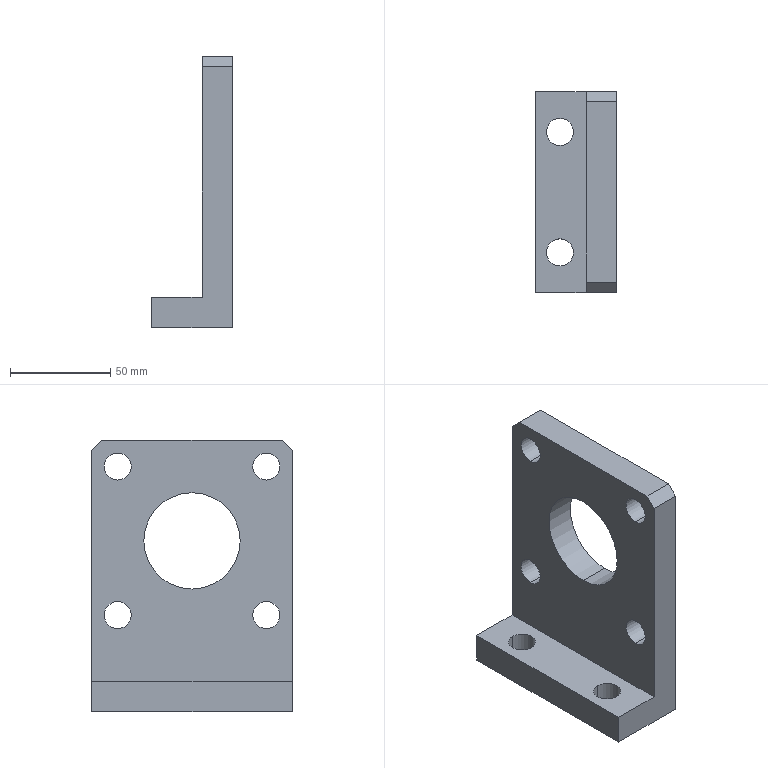Component | SolidWorks | ZN-A-012-1 | 1 solid | 24 faces | box 40 x 100 x 135 mm | volume 199599 mm3 | cylinder 14 | plane 10 | commonest cylinder face diameters 13.5 x12 48 x2
build123d program:
from build123d import *

# Parameters (mm, degrees)
SKETCH1_W                 = 100
SKETCH1_H                 = 135
BOSS_EXTRUDE1_DEPTH       = 7.5
SKETCH2_W                 = 15
SKETCH2_H                 = 25
BOSS_EXTRUDE2_DEPTH       = 100
SKETCH3_R                 = 24
CUT_EXTRUDE1_DEPTH        = 94.039
M12_CLEARANCE_HOLE1_D     = 13.5
M12_CLEARANCE_HOLE1_DEPTH = 15
M12_CLEARANCE_HOLE1_TIP   = 4.056
M12_CLEARANCE_HOLE2_D     = 13.5
M12_CLEARANCE_HOLE2_DEPTH = 15
M12_CLEARANCE_HOLE2_TIP   = 4.056
CHAMFER1_SIZE             = 5


with BuildPart() as part:
    # Sketch1 → Boss-Extrude1 (new, symmetric)
    with BuildSketch(Plane(origin=(0, 0, 0), x_dir=(1, 0, 0), z_dir=(0, 1, 0))):
        Rectangle(SKETCH1_W, SKETCH1_H)
    extrude(amount=BOSS_EXTRUDE1_DEPTH, both=True)

    # Sketch2 → Boss-Extrude2 (add)
    with BuildSketch(Plane.ZY.offset(50)):
        with Locations((60, 20)):
            Rectangle(SKETCH2_W, SKETCH2_H)
    extrude(amount=-BOSS_EXTRUDE2_DEPTH)

    # Sketch3 → Cut-Extrude1 (cut, through all)
    with BuildSketch(Plane.XZ.offset(7.5)):
        with Locations(Location((0, -17.5, 0), (0, 0, 270))):
            Circle(SKETCH3_R)
    extrude(amount=-CUT_EXTRUDE1_DEPTH, mode=Mode.SUBTRACT)

    # M12 Clearance Hole1
    with Locations(Plane(origin=(0, 7.5, 0), x_dir=(1, 0, 0), z_dir=(0, 1, 0))):
        with Locations((-37, 54.5), (37, 54.5), (-37, -19.5), (37, -19.5)):
            Hole(M12_CLEARANCE_HOLE1_D / 2, depth=M12_CLEARANCE_HOLE1_DEPTH)
            with Locations((0, 0, -(M12_CLEARANCE_HOLE1_DEPTH + M12_CLEARANCE_HOLE1_TIP / 2))):  # 118° drill point
                Cone(0, M12_CLEARANCE_HOLE1_D / 2, M12_CLEARANCE_HOLE1_TIP, mode=Mode.SUBTRACT)

    # M12 Clearance Hole2
    with Locations(Plane(origin=(0, 0, 52.5), x_dir=(-1, 0, 0), z_dir=(0, 0, -1))):
        with Locations((-30, 20.5), (30, 20.5)):
            Hole(M12_CLEARANCE_HOLE2_D / 2, depth=M12_CLEARANCE_HOLE2_DEPTH)
            with Locations((0, 0, -(M12_CLEARANCE_HOLE2_DEPTH + M12_CLEARANCE_HOLE2_TIP / 2))):  # 118° drill point
                Cone(0, M12_CLEARANCE_HOLE2_D / 2, M12_CLEARANCE_HOLE2_TIP, mode=Mode.SUBTRACT)

    # Chamfer1
    chamfer1_edges = [part.edges().sort_by_distance(p)[0] for p in [
        (50, 0, -67.5),
        (-50, 0, -67.5),
    ]]
    chamfer(chamfer1_edges, length=CHAMFER1_SIZE)


solid = part.part

# Placed as in the assembly
solid = solid.moved(Location((640.892, 232.499, 82.5), (180, 0, 90)))
STEP:
#1=CARTESIAN_POINT('',(24.425,7.707,0.5906));
#2=VERTEX_POINT('',#1);
#3=CARTESIAN_POINT('',(24.425,8.238,0.5906));
#4=VERTEX_POINT('',#3);
#5=CARTESIAN_POINT('',(24.425,7.972,0.5906));
#6=DIRECTION('',(-0.,-0.,1.));
#7=DIRECTION('',(0.,1.,0.));
#8=AXIS2_PLACEMENT_3D('',#5,#6,#7);
#9=CIRCLE('',#8,0.2657);
#10=EDGE_CURVE('',#2,#4,#9,.T.);
#11=ORIENTED_EDGE('',*,*,#10,.F.);
#12=CARTESIAN_POINT('',(24.425,7.707,1.181));
#13=VERTEX_POINT('',#12);
#14=CARTESIAN_POINT('',(24.425,7.707,1.181));
#15=DIRECTION('',(-0.,-0.,1.));
#16=VECTOR('',#15,39.37);
#17=LINE('',#14,#16);
#18=EDGE_CURVE('',#2,#13,#17,.T.);
#19=ORIENTED_EDGE('',*,*,#18,.T.);
#20=CARTESIAN_POINT('',(24.425,8.238,1.181));
#21=VERTEX_POINT('',#20);
#22=CARTESIAN_POINT('',(24.425,7.972,1.181));
#23=DIRECTION('',(-0.,-0.,1.));
#24=DIRECTION('',(0.,1.,0.));
#25=AXIS2_PLACEMENT_3D('',#22,#23,#24);
#26=CIRCLE('',#25,0.2657);
#27=EDGE_CURVE('',#13,#21,#26,.T.);
#28=ORIENTED_EDGE('',*,*,#27,.T.);
#29=CARTESIAN_POINT('',(24.425,8.238,1.181));
#30=DIRECTION('',(-0.,-0.,1.));
#31=VECTOR('',#30,39.37);
#32=LINE('',#29,#31);
#33=EDGE_CURVE('',#4,#21,#32,.T.);
#34=ORIENTED_EDGE('',*,*,#33,.F.);
#35=EDGE_LOOP('',(#11,#19,#28,#34));
#36=FACE_OUTER_BOUND('',#35,.T.);
#37=CARTESIAN_POINT('',(24.425,7.972,1.181));
#38=DIRECTION('',(-0.,-0.,1.));
#39=DIRECTION('',(0.,1.,0.));
#40=AXIS2_PLACEMENT_3D('',#37,#38,#39);
#41=CYLINDRICAL_SURFACE('',#40,0.2657);
#42=ADVANCED_FACE('',(#36),#41,.F.);
#43=CARTESIAN_POINT('',(24.425,10.069,0.5906));
#44=VERTEX_POINT('',#43);
#45=CARTESIAN_POINT('',(24.425,10.6,0.5906));
#46=VERTEX_POINT('',#45);
#47=CARTESIAN_POINT('',(24.425,10.335,0.5906));
#48=DIRECTION('',(-0.,-0.,1.));
#49=DIRECTION('',(0.,1.,0.));
#50=AXIS2_PLACEMENT_3D('',#47,#48,#49);
#51=CIRCLE('',#50,0.2657);
#52=EDGE_CURVE('',#44,#46,#51,.T.);
#53=ORIENTED_EDGE('',*,*,#52,.F.);
#54=CARTESIAN_POINT('',(24.425,10.069,1.181));
#55=VERTEX_POINT('',#54);
#56=CARTESIAN_POINT('',(24.425,10.069,1.181));
#57=DIRECTION('',(-0.,-0.,1.));
#58=VECTOR('',#57,39.37);
#59=LINE('',#56,#58);
#60=EDGE_CURVE('',#44,#55,#59,.T.);
#61=ORIENTED_EDGE('',*,*,#60,.T.);
#62=CARTESIAN_POINT('',(24.425,10.6,1.181));
#63=VERTEX_POINT('',#62);
#64=CARTESIAN_POINT('',(24.425,10.335,1.181));
#65=DIRECTION('',(-0.,-0.,1.));
#66=DIRECTION('',(0.,1.,0.));
#67=AXIS2_PLACEMENT_3D('',#64,#65,#66);
#68=CIRCLE('',#67,0.2657);
#69=EDGE_CURVE('',#55,#63,#68,.T.);
#70=ORIENTED_EDGE('',*,*,#69,.T.);
#71=CARTESIAN_POINT('',(24.425,10.6,1.181));
#72=DIRECTION('',(-0.,-0.,1.));
#73=VECTOR('',#72,39.37);
#74=LINE('',#71,#73);
#75=EDGE_CURVE('',#46,#63,#74,.T.);
#76=ORIENTED_EDGE('',*,*,#75,.F.);
#77=EDGE_LOOP('',(#53,#61,#70,#76));
#78=FACE_OUTER_BOUND('',#77,.T.);
#79=CARTESIAN_POINT('',(24.425,10.335,1.181));
#80=DIRECTION('',(-0.,-0.,1.));
#81=DIRECTION('',(0.,1.,0.));
#82=AXIS2_PLACEMENT_3D('',#79,#80,#81);
#83=CYLINDRICAL_SURFACE('',#82,0.2657);
#84=ADVANCED_FACE('',(#78),#83,.F.);
#85=CARTESIAN_POINT('',(25.527,10.61,5.659));
#86=VERTEX_POINT('',#85);
#87=CARTESIAN_POINT('',(25.527,10.61,5.128));
#88=VERTEX_POINT('',#87);
#89=CARTESIAN_POINT('',(25.527,10.61,5.394));
#90=DIRECTION('',(-1.,-0.,-0.));
#91=DIRECTION('',(0.,0.,-1.));
#92=AXIS2_PLACEMENT_3D('',#89,#90,#91);
#93=CIRCLE('',#92,0.2657);
#94=EDGE_CURVE('',#86,#88,#93,.T.);
#95=ORIENTED_EDGE('',*,*,#94,.F.);
#96=CARTESIAN_POINT('',(24.937,10.61,5.659));
#97=VERTEX_POINT('',#96);
#98=CARTESIAN_POINT('',(24.937,10.61,5.659));
#99=DIRECTION('',(-1.,-0.,-0.));
#100=VECTOR('',#99,39.37);
#101=LINE('',#98,#100);
#102=EDGE_CURVE('',#86,#97,#101,.T.);
#103=ORIENTED_EDGE('',*,*,#102,.T.);
#104=CARTESIAN_POINT('',(24.937,10.61,5.128));
#105=VERTEX_POINT('',#104);
#106=CARTESIAN_POINT('',(24.937,10.61,5.394));
#107=DIRECTION('',(-1.,-0.,-0.));
#108=DIRECTION('',(0.,0.,-1.));
#109=AXIS2_PLACEMENT_3D('',#106,#107,#108);
#110=CIRCLE('',#109,0.2657);
#111=EDGE_CURVE('',#97,#105,#110,.T.);
#112=ORIENTED_EDGE('',*,*,#111,.T.);
#113=CARTESIAN_POINT('',(24.937,10.61,5.128));
#114=DIRECTION('',(-1.,-0.,-0.));
#115=VECTOR('',#114,39.37);
#116=LINE('',#113,#115);
#117=EDGE_CURVE('',#88,#105,#116,.T.);
#118=ORIENTED_EDGE('',*,*,#117,.F.);
#119=EDGE_LOOP('',(#95,#103,#112,#118));
#120=FACE_OUTER_BOUND('',#119,.T.);
#121=CARTESIAN_POINT('',(24.937,10.61,5.394));
#122=DIRECTION('',(-1.,-0.,-0.));
#123=DIRECTION('',(0.,0.,-1.));
#124=AXIS2_PLACEMENT_3D('',#121,#122,#123);
#125=CYLINDRICAL_SURFACE('',#124,0.2657);
#126=ADVANCED_FACE('',(#120),#125,.F.);
#127=CARTESIAN_POINT('',(25.527,7.697,5.659));
#128=VERTEX_POINT('',#127);
#129=CARTESIAN_POINT('',(25.527,7.697,5.128));
#130=VERTEX_POINT('',#129);
#131=CARTESIAN_POINT('',(25.527,7.697,5.394));
#132=DIRECTION('',(-1.,-0.,-0.));
#133=DIRECTION('',(0.,0.,-1.));
#134=AXIS2_PLACEMENT_3D('',#131,#132,#133);
#135=CIRCLE('',#134,0.2657);
#136=EDGE_CURVE('',#128,#130,#135,.T.);
#137=ORIENTED_EDGE('',*,*,#136,.F.);
#138=CARTESIAN_POINT('',(24.937,7.697,5.659));
#139=VERTEX_POINT('',#138);
#140=CARTESIAN_POINT('',(24.937,7.697,5.659));
#141=DIRECTION('',(-1.,-0.,-0.));
#142=VECTOR('',#141,39.37);
#143=LINE('',#140,#142);
#144=EDGE_CURVE('',#128,#139,#143,.T.);
#145=ORIENTED_EDGE('',*,*,#144,.T.);
#146=CARTESIAN_POINT('',(24.937,7.697,5.128));
#147=VERTEX_POINT('',#146);
#148=CARTESIAN_POINT('',(24.937,7.697,5.394));
#149=DIRECTION('',(-1.,-0.,-0.));
#150=DIRECTION('',(0.,0.,-1.));
#151=AXIS2_PLACEMENT_3D('',#148,#149,#150);
#152=CIRCLE('',#151,0.2657);
#153=EDGE_CURVE('',#139,#147,#152,.T.);
#154=ORIENTED_EDGE('',*,*,#153,.T.);
#155=CARTESIAN_POINT('',(24.937,7.697,5.128));
#156=DIRECTION('',(-1.,-0.,-0.));
#157=VECTOR('',#156,39.37);
#158=LINE('',#155,#157);
#159=EDGE_CURVE('',#130,#147,#158,.T.);
#160=ORIENTED_EDGE('',*,*,#159,.F.);
#161=EDGE_LOOP('',(#137,#145,#154,#160));
#162=FACE_OUTER_BOUND('',#161,.T.);
#163=CARTESIAN_POINT('',(24.937,7.697,5.394));
#164=DIRECTION('',(-1.,-0.,-0.));
#165=DIRECTION('',(0.,0.,-1.));
#166=AXIS2_PLACEMENT_3D('',#163,#164,#165);
#167=CYLINDRICAL_SURFACE('',#166,0.2657);
#168=ADVANCED_FACE('',(#162),#167,.F.);
#169=CARTESIAN_POINT('',(25.527,10.61,2.746));
#170=VERTEX_POINT('',#169);
#171=CARTESIAN_POINT('',(25.527,10.61,2.215));
#172=VERTEX_POINT('',#171);
#173=CARTESIAN_POINT('',(25.527,10.61,2.48));
#174=DIRECTION('',(-1.,-0.,-0.));
#175=DIRECTION('',(0.,0.,-1.));
#176=AXIS2_PLACEMENT_3D('',#173,#174,#175);
#177=CIRCLE('',#176,0.2657);
#178=EDGE_CURVE('',#170,#172,#177,.T.);
#179=ORIENTED_EDGE('',*,*,#178,.F.);
#180=CARTESIAN_POINT('',(24.937,10.61,2.746));
#181=VERTEX_POINT('',#180);
#182=CARTESIAN_POINT('',(24.937,10.61,2.746));
#183=DIRECTION('',(-1.,-0.,-0.));
#184=VECTOR('',#183,39.37);
#185=LINE('',#182,#184);
#186=EDGE_CURVE('',#170,#181,#185,.T.);
#187=ORIENTED_EDGE('',*,*,#186,.T.);
#188=CARTESIAN_POINT('',(24.937,10.61,2.215));
#189=VERTEX_POINT('',#188);
#190=CARTESIAN_POINT('',(24.937,10.61,2.48));
#191=DIRECTION('',(-1.,-0.,-0.));
#192=DIRECTION('',(0.,0.,-1.));
#193=AXIS2_PLACEMENT_3D('',#190,#191,#192);
#194=CIRCLE('',#193,0.2657);
#195=EDGE_CURVE('',#181,#189,#194,.T.);
#196=ORIENTED_EDGE('',*,*,#195,.T.);
#197=CARTESIAN_POINT('',(24.937,10.61,2.215));
#198=DIRECTION('',(-1.,-0.,-0.));
#199=VECTOR('',#198,39.37);
#200=LINE('',#197,#199);
#201=EDGE_CURVE('',#172,#189,#200,.T.);
#202=ORIENTED_EDGE('',*,*,#201,.F.);
#203=EDGE_LOOP('',(#179,#187,#196,#202));
#204=FACE_OUTER_BOUND('',#203,.T.);
#205=CARTESIAN_POINT('',(24.937,10.61,2.48));
#206=DIRECTION('',(-1.,-0.,-0.));
#207=DIRECTION('',(0.,0.,-1.));
#208=AXIS2_PLACEMENT_3D('',#205,#206,#207);
#209=CYLINDRICAL_SURFACE('',#208,0.2657);
#210=ADVANCED_FACE('',(#204),#209,.F.);
#211=CARTESIAN_POINT('',(25.527,7.697,2.746));
#212=VERTEX_POINT('',#211);
#213=CARTESIAN_POINT('',(25.527,7.697,2.215));
#214=VERTEX_POINT('',#213);
#215=CARTESIAN_POINT('',(25.527,7.697,2.48));
#216=DIRECTION('',(-1.,-0.,-0.));
#217=DIRECTION('',(0.,0.,-1.));
#218=AXIS2_PLACEMENT_3D('',#215,#216,#217);
#219=CIRCLE('',#218,0.2657);
#220=EDGE_CURVE('',#212,#214,#219,.T.);
#221=ORIENTED_EDGE('',*,*,#220,.F.);
#222=CARTESIAN_POINT('',(24.937,7.697,2.746));
#223=VERTEX_POINT('',#222);
#224=CARTESIAN_POINT('',(24.937,7.697,2.746));
#225=DIRECTION('',(-1.,-0.,-0.));
#226=VECTOR('',#225,39.37);
#227=LINE('',#224,#226);
#228=EDGE_CURVE('',#212,#223,#227,.T.);
#229=ORIENTED_EDGE('',*,*,#228,.T.);
#230=CARTESIAN_POINT('',(24.937,7.697,2.215));
#231=VERTEX_POINT('',#230);
#232=CARTESIAN_POINT('',(24.937,7.697,2.48));
#233=DIRECTION('',(-1.,-0.,-0.));
#234=DIRECTION('',(0.,0.,-1.));
#235=AXIS2_PLACEMENT_3D('',#232,#233,#234);
#236=CIRCLE('',#235,0.2657);
#237=EDGE_CURVE('',#223,#231,#236,.T.);
#238=ORIENTED_EDGE('',*,*,#237,.T.);
#239=CARTESIAN_POINT('',(24.937,7.697,2.215));
#240=DIRECTION('',(-1.,-0.,-0.));
#241=VECTOR('',#240,39.37);
#242=LINE('',#239,#241);
#243=EDGE_CURVE('',#214,#231,#242,.T.);
#244=ORIENTED_EDGE('',*,*,#243,.F.);
#245=EDGE_LOOP('',(#221,#229,#238,#244));
#246=FACE_OUTER_BOUND('',#245,.T.);
#247=CARTESIAN_POINT('',(24.937,7.697,2.48));
#248=DIRECTION('',(-1.,-0.,-0.));
#249=DIRECTION('',(0.,0.,-1.));
#250=AXIS2_PLACEMENT_3D('',#247,#248,#249);
#251=CYLINDRICAL_SURFACE('',#250,0.2657);
#252=ADVANCED_FACE('',(#246),#251,.F.);
#253=CARTESIAN_POINT('',(24.937,9.154,4.882));
#254=VERTEX_POINT('',#253);
#255=CARTESIAN_POINT('',(24.937,9.154,2.992));
#256=VERTEX_POINT('',#255);
#257=CARTESIAN_POINT('',(24.937,9.154,3.937));
#258=DIRECTION('',(-1.,-0.,-0.));
#259=DIRECTION('',(0.,0.,-1.));
#260=AXIS2_PLACEMENT_3D('',#257,#258,#259);
#261=CIRCLE('',#260,0.9449);
#262=EDGE_CURVE('',#254,#256,#261,.T.);
#263=ORIENTED_EDGE('',*,*,#262,.T.);
#264=CARTESIAN_POINT('',(25.527,9.154,2.992));
#265=VERTEX_POINT('',#264);
#266=CARTESIAN_POINT('',(23.952,9.154,2.992));
#267=DIRECTION('',(1.,0.,0.));
#268=VECTOR('',#267,39.37);
#269=LINE('',#266,#268);
#270=EDGE_CURVE('',#256,#265,#269,.T.);
#271=ORIENTED_EDGE('',*,*,#270,.T.);
#272=CARTESIAN_POINT('',(25.527,9.154,4.882));
#273=VERTEX_POINT('',#272);
#274=CARTESIAN_POINT('',(25.527,9.154,3.937));
#275=DIRECTION('',(1.,0.,0.));
#276=DIRECTION('',(0.,-0.,1.));
#277=AXIS2_PLACEMENT_3D('',#274,#275,#276);
#278=CIRCLE('',#277,0.9449);
#279=EDGE_CURVE('',#265,#273,#278,.T.);
#280=ORIENTED_EDGE('',*,*,#279,.T.);
#281=CARTESIAN_POINT('',(23.952,9.154,4.882));
#282=DIRECTION('',(1.,0.,0.));
#283=VECTOR('',#282,39.37);
#284=LINE('',#281,#283);
#285=EDGE_CURVE('',#254,#273,#284,.T.);
#286=ORIENTED_EDGE('',*,*,#285,.F.);
#287=EDGE_LOOP('',(#263,#271,#280,#286));
#288=FACE_OUTER_BOUND('',#287,.T.);
#289=CARTESIAN_POINT('',(23.952,9.154,3.937));
#290=DIRECTION('',(1.,0.,0.));
#291=DIRECTION('',(0.,-0.,1.));
#292=AXIS2_PLACEMENT_3D('',#289,#290,#291);
#293=CYLINDRICAL_SURFACE('',#292,0.9449);
#294=ADVANCED_FACE('',(#288),#293,.F.);
#295=CARTESIAN_POINT('',(24.937,11.122,5.709));
#296=VERTEX_POINT('',#295);
#297=CARTESIAN_POINT('',(24.937,11.122,1.181));
#298=VERTEX_POINT('',#297);
#299=CARTESIAN_POINT('',(24.937,11.122,5.906));
#300=DIRECTION('',(0.,0.,-1.));
#301=VECTOR('',#300,39.37);
#302=LINE('',#299,#301);
#303=EDGE_CURVE('',#296,#298,#302,.T.);
#304=ORIENTED_EDGE('',*,*,#303,.F.);
#305=CARTESIAN_POINT('',(25.527,11.122,5.709));
#306=VERTEX_POINT('',#305);
#307=CARTESIAN_POINT('',(24.937,11.122,5.709));
#308=DIRECTION('',(1.,0.,0.));
#309=VECTOR('',#308,39.37);
#310=LINE('',#307,#309);
#311=EDGE_CURVE('',#296,#306,#310,.T.);
#312=ORIENTED_EDGE('',*,*,#311,.T.);
#313=CARTESIAN_POINT('',(25.527,11.122,0.5906));
#314=VERTEX_POINT('',#313);
#315=CARTESIAN_POINT('',(25.527,11.122,5.906));
#316=DIRECTION('',(0.,0.,-1.));
#317=VECTOR('',#316,39.37);
#318=LINE('',#315,#317);
#319=EDGE_CURVE('',#306,#314,#318,.T.);
#320=ORIENTED_EDGE('',*,*,#319,.T.);
#321=CARTESIAN_POINT('',(23.952,11.122,0.5906));
#322=VERTEX_POINT('',#321);
#323=CARTESIAN_POINT('',(24.937,11.122,0.5906));
#324=DIRECTION('',(1.,0.,0.));
#325=VECTOR('',#324,39.37);
#326=LINE('',#323,#325);
#327=EDGE_CURVE('',#322,#314,#326,.T.);
#328=ORIENTED_EDGE('',*,*,#327,.F.);
#329=CARTESIAN_POINT('',(23.952,11.122,1.181));
#330=VERTEX_POINT('',#329);
#331=CARTESIAN_POINT('',(23.952,11.122,0.5906));
#332=DIRECTION('',(-0.,-0.,1.));
#333=VECTOR('',#332,39.37);
#334=LINE('',#331,#333);
#335=EDGE_CURVE('',#322,#330,#334,.T.);
#336=ORIENTED_EDGE('',*,*,#335,.T.);
#337=CARTESIAN_POINT('',(24.937,11.122,1.181));
#338=DIRECTION('',(1.,0.,0.));
#339=VECTOR('',#338,39.37);
#340=LINE('',#337,#339);
#341=EDGE_CURVE('',#330,#298,#340,.T.);
#342=ORIENTED_EDGE('',*,*,#341,.T.);
#343=EDGE_LOOP('',(#304,#312,#320,#328,#336,#342));
#344=FACE_OUTER_BOUND('',#343,.T.);
#345=CARTESIAN_POINT('',(24.937,11.122,5.906));
#346=DIRECTION('',(0.,-1.,-0.));
#347=DIRECTION('',(-0.,-0.,1.));
#348=AXIS2_PLACEMENT_3D('',#345,#346,#347);
#349=PLANE('',#348);
#350=ADVANCED_FACE('',(#344),#349,.F.);
#351=CARTESIAN_POINT('',(24.425,7.972,0.5906));
#352=DIRECTION('',(-0.,-0.,1.));
#353=DIRECTION('',(0.,1.,0.));
#354=AXIS2_PLACEMENT_3D('',#351,#352,#353);
#355=CIRCLE('',#354,0.2657);
#356=EDGE_CURVE('',#4,#2,#355,.T.);
#357=ORIENTED_EDGE('',*,*,#356,.T.);
#358=ORIENTED_EDGE('',*,*,#10,.T.);
#359=EDGE_LOOP('',(#357,#358));
#360=FACE_BOUND('',#359,.T.);
#361=CARTESIAN_POINT('',(24.425,10.335,0.5906));
#362=DIRECTION('',(-0.,-0.,1.));
#363=DIRECTION('',(0.,1.,0.));
#364=AXIS2_PLACEMENT_3D('',#361,#362,#363);
#365=CIRCLE('',#364,0.2657);
#366=EDGE_CURVE('',#46,#44,#365,.T.);
#367=ORIENTED_EDGE('',*,*,#366,.T.);
#368=ORIENTED_EDGE('',*,*,#52,.T.);
#369=EDGE_LOOP('',(#367,#368));
#370=FACE_BOUND('',#369,.T.);
#371=CARTESIAN_POINT('',(25.527,7.185,0.5906));
#372=VERTEX_POINT('',#371);
#373=CARTESIAN_POINT('',(25.527,11.122,0.5906));
#374=DIRECTION('',(0.,-1.,-0.));
#375=VECTOR('',#374,39.37);
#376=LINE('',#373,#375);
#377=EDGE_CURVE('',#314,#372,#376,.T.);
#378=ORIENTED_EDGE('',*,*,#377,.T.);
#379=CARTESIAN_POINT('',(23.952,7.185,0.5906));
#380=VERTEX_POINT('',#379);
#381=CARTESIAN_POINT('',(24.937,7.185,0.5906));
#382=DIRECTION('',(1.,0.,0.));
#383=VECTOR('',#382,39.37);
#384=LINE('',#381,#383);
#385=EDGE_CURVE('',#380,#372,#384,.T.);
#386=ORIENTED_EDGE('',*,*,#385,.F.);
#387=CARTESIAN_POINT('',(23.952,7.185,0.5906));
#388=DIRECTION('',(-0.,1.,0.));
#389=VECTOR('',#388,39.37);
#390=LINE('',#387,#389);
#391=EDGE_CURVE('',#380,#322,#390,.T.);
#392=ORIENTED_EDGE('',*,*,#391,.T.);
#393=ORIENTED_EDGE('',*,*,#327,.T.);
#394=EDGE_LOOP('',(#378,#386,#392,#393));
#395=FACE_OUTER_BOUND('',#394,.T.);
#396=CARTESIAN_POINT('',(24.937,11.122,0.5906));
#397=DIRECTION('',(-0.,-0.,1.));
#398=DIRECTION('',(-0.,1.,0.));
#399=AXIS2_PLACEMENT_3D('',#396,#397,#398);
#400=PLANE('',#399);
#401=ADVANCED_FACE('',(#360,#370,#395),#400,.F.);
#402=CARTESIAN_POINT('',(25.527,7.185,5.709));
#403=VERTEX_POINT('',#402);
#404=CARTESIAN_POINT('',(25.527,7.185,5.906));
#405=DIRECTION('',(-0.,-0.,1.));
#406=VECTOR('',#405,39.37);
#407=LINE('',#404,#406);
#408=EDGE_CURVE('',#372,#403,#407,.T.);
#409=ORIENTED_EDGE('',*,*,#408,.T.);
#410=CARTESIAN_POINT('',(24.937,7.185,5.709));
#411=VERTEX_POINT('',#410);
#412=CARTESIAN_POINT('',(24.937,7.185,5.709));
#413=DIRECTION('',(-1.,-0.,-0.));
#414=VECTOR('',#413,39.37);
#415=LINE('',#412,#414);
#416=EDGE_CURVE('',#403,#411,#415,.T.);
#417=ORIENTED_EDGE('',*,*,#416,.T.);
#418=CARTESIAN_POINT('',(24.937,7.185,1.181));
#419=VERTEX_POINT('',#418);
#420=CARTESIAN_POINT('',(24.937,7.185,5.906));
#421=DIRECTION('',(-0.,-0.,1.));
#422=VECTOR('',#421,39.37);
#423=LINE('',#420,#422);
#424=EDGE_CURVE('',#419,#411,#423,.T.);
#425=ORIENTED_EDGE('',*,*,#424,.F.);
#426=CARTESIAN_POINT('',(23.952,7.185,1.181));
#427=VERTEX_POINT('',#426);
#428=CARTESIAN_POINT('',(24.937,7.185,1.181));
#429=DIRECTION('',(1.,0.,0.));
#430=VECTOR('',#429,39.37);
#431=LINE('',#428,#430);
#432=EDGE_CURVE('',#427,#419,#431,.T.);
#433=ORIENTED_EDGE('',*,*,#432,.F.);
#434=CARTESIAN_POINT('',(23.952,7.185,0.5906));
#435=DIRECTION('',(-0.,-0.,1.));
#436=VECTOR('',#435,39.37);
#437=LINE('',#434,#436);
#438=EDGE_CURVE('',#380,#427,#437,.T.);
#439=ORIENTED_EDGE('',*,*,#438,.F.);
#440=ORIENTED_EDGE('',*,*,#385,.T.);
#441=EDGE_LOOP('',(#409,#417,#425,#433,#439,#440));
#442=FACE_OUTER_BOUND('',#441,.T.);
#443=CARTESIAN_POINT('',(24.937,7.185,5.906));
#444=DIRECTION('',(-0.,1.,0.));
#445=DIRECTION('',(0.,0.,-1.));
#446=AXIS2_PLACEMENT_3D('',#443,#444,#445);
#447=PLANE('',#446);
#448=ADVANCED_FACE('',(#442),#447,.F.);
#449=CARTESIAN_POINT('',(24.937,7.382,5.906));
#450=VERTEX_POINT('',#449);
#451=CARTESIAN_POINT('',(24.937,10.925,5.906));
#452=VERTEX_POINT('',#451);
#453=CARTESIAN_POINT('',(24.937,11.122,5.906));
#454=DIRECTION('',(-0.,1.,0.));
#455=VECTOR('',#454,39.37);
#456=LINE('',#453,#455);
#457=EDGE_CURVE('',#450,#452,#456,.T.);
#458=ORIENTED_EDGE('',*,*,#457,.F.);
#459=CARTESIAN_POINT('',(25.527,7.382,5.906));
#460=VERTEX_POINT('',#459);
#461=CARTESIAN_POINT('',(24.937,7.382,5.906));
#462=DIRECTION('',(1.,0.,0.));
#463=VECTOR('',#462,39.37);
#464=LINE('',#461,#463);
#465=EDGE_CURVE('',#450,#460,#464,.T.);
#466=ORIENTED_EDGE('',*,*,#465,.T.);
#467=CARTESIAN_POINT('',(25.527,10.925,5.906));
#468=VERTEX_POINT('',#467);
#469=CARTESIAN_POINT('',(25.527,11.122,5.906));
#470=DIRECTION('',(-0.,1.,0.));
#471=VECTOR('',#470,39.37);
#472=LINE('',#469,#471);
#473=EDGE_CURVE('',#460,#468,#472,.T.);
#474=ORIENTED_EDGE('',*,*,#473,.T.);
#475=CARTESIAN_POINT('',(24.937,10.925,5.906));
#476=DIRECTION('',(-1.,-0.,-0.));
#477=VECTOR('',#476,39.37);
#478=LINE('',#475,#477);
#479=EDGE_CURVE('',#468,#452,#478,.T.);
#480=ORIENTED_EDGE('',*,*,#479,.T.);
#481=EDGE_LOOP('',(#458,#466,#474,#480));
#482=FACE_OUTER_BOUND('',#481,.T.);
#483=CARTESIAN_POINT('',(24.937,11.122,5.906));
#484=DIRECTION('',(0.,0.,-1.));
#485=DIRECTION('',(0.,-1.,-0.));
#486=AXIS2_PLACEMENT_3D('',#483,#484,#485);
#487=PLANE('',#486);
#488=ADVANCED_FACE('',(#482),#487,.F.);
#489=CARTESIAN_POINT('',(24.937,10.61,5.394));
#490=DIRECTION('',(-1.,-0.,-0.));
#491=DIRECTION('',(0.,0.,-1.));
#492=AXIS2_PLACEMENT_3D('',#489,#490,#491);
#493=CIRCLE('',#492,0.2657);
#494=EDGE_CURVE('',#105,#97,#493,.T.);
#495=ORIENTED_EDGE('',*,*,#494,.F.);
#496=ORIENTED_EDGE('',*,*,#111,.F.);
#497=EDGE_LOOP('',(#495,#496));
#498=FACE_BOUND('',#497,.T.);
#499=CARTESIAN_POINT('',(24.937,7.697,5.394));
#500=DIRECTION('',(-1.,-0.,-0.));
#501=DIRECTION('',(0.,0.,-1.));
#502=AXIS2_PLACEMENT_3D('',#499,#500,#501);
#503=CIRCLE('',#502,0.2657);
#504=EDGE_CURVE('',#147,#139,#503,.T.);
#505=ORIENTED_EDGE('',*,*,#504,.F.);
#506=ORIENTED_EDGE('',*,*,#153,.F.);
#507=EDGE_LOOP('',(#505,#506));
#508=FACE_BOUND('',#507,.T.);
#509=CARTESIAN_POINT('',(24.937,10.61,2.48));
#510=DIRECTION('',(-1.,-0.,-0.));
#511=DIRECTION('',(0.,0.,-1.));
#512=AXIS2_PLACEMENT_3D('',#509,#510,#511);
#513=CIRCLE('',#512,0.2657);
#514=EDGE_CURVE('',#189,#181,#513,.T.);
#515=ORIENTED_EDGE('',*,*,#514,.F.);
#516=ORIENTED_EDGE('',*,*,#195,.F.);
#517=EDGE_LOOP('',(#515,#516));
#518=FACE_BOUND('',#517,.T.);
#519=CARTESIAN_POINT('',(24.937,7.697,2.48));
#520=DIRECTION('',(-1.,-0.,-0.));
#521=DIRECTION('',(0.,0.,-1.));
#522=AXIS2_PLACEMENT_3D('',#519,#520,#521);
#523=CIRCLE('',#522,0.2657);
#524=EDGE_CURVE('',#231,#223,#523,.T.);
#525=ORIENTED_EDGE('',*,*,#524,.F.);
#526=ORIENTED_EDGE('',*,*,#237,.F.);
#527=EDGE_LOOP('',(#525,#526));
#528=FACE_BOUND('',#527,.T.);
#529=ORIENTED_EDGE('',*,*,#262,.F.);
#530=CARTESIAN_POINT('',(24.937,9.154,3.937));
#531=DIRECTION('',(-1.,-0.,-0.));
#532=DIRECTION('',(0.,0.,-1.));
#533=AXIS2_PLACEMENT_3D('',#530,#531,#532);
#534=CIRCLE('',#533,0.9449);
#535=EDGE_CURVE('',#256,#254,#534,.T.);
#536=ORIENTED_EDGE('',*,*,#535,.F.);
#537=EDGE_LOOP('',(#529,#536));
#538=FACE_BOUND('',#537,.T.);
#539=ORIENTED_EDGE('',*,*,#424,.T.);
#540=CARTESIAN_POINT('',(24.937,6.594,5.118));
#541=DIRECTION('',(-0.,0.7071,0.7071));
#542=VECTOR('',#541,39.37);
#543=LINE('',#540,#542);
#544=EDGE_CURVE('',#411,#450,#543,.T.);
#545=ORIENTED_EDGE('',*,*,#544,.T.);
#546=ORIENTED_EDGE('',*,*,#457,.T.);
#547=CARTESIAN_POINT('',(24.937,13.681,3.15));
#548=DIRECTION('',(0.,0.7071,-0.7071));
#549=VECTOR('',#548,39.37);
#550=LINE('',#547,#549);
#551=EDGE_CURVE('',#452,#296,#550,.T.);
#552=ORIENTED_EDGE('',*,*,#551,.T.);
#553=ORIENTED_EDGE('',*,*,#303,.T.);
#554=CARTESIAN_POINT('',(24.937,7.185,1.181));
#555=DIRECTION('',(-0.,1.,0.));
#556=VECTOR('',#555,39.37);
#557=LINE('',#554,#556);
#558=EDGE_CURVE('',#419,#298,#557,.T.);
#559=ORIENTED_EDGE('',*,*,#558,.F.);
#560=EDGE_LOOP('',(#539,#545,#546,#552,#553,#559));
#561=FACE_OUTER_BOUND('',#560,.T.);
#562=CARTESIAN_POINT('',(24.937,11.122,0.5906));
#563=DIRECTION('',(-1.,-0.,-0.));
#564=DIRECTION('',(0.,0.,-1.));
#565=AXIS2_PLACEMENT_3D('',#562,#563,#564);
#566=PLANE('',#565);
#567=ADVANCED_FACE('',(#498,#508,#518,#528,#538,#561),#566,.T.);
#568=CARTESIAN_POINT('',(25.527,10.61,5.394));
#569=DIRECTION('',(-1.,-0.,-0.));
#570=DIRECTION('',(0.,0.,-1.));
#571=AXIS2_PLACEMENT_3D('',#568,#569,#570);
#572=CIRCLE('',#571,0.2657);
#573=EDGE_CURVE('',#88,#86,#572,.T.);
#574=ORIENTED_EDGE('',*,*,#573,.T.);
#575=ORIENTED_EDGE('',*,*,#94,.T.);
#576=EDGE_LOOP('',(#574,#575));
#577=FACE_BOUND('',#576,.T.);
#578=CARTESIAN_POINT('',(25.527,7.697,5.394));
#579=DIRECTION('',(-1.,-0.,-0.));
#580=DIRECTION('',(0.,0.,-1.));
#581=AXIS2_PLACEMENT_3D('',#578,#579,#580);
#582=CIRCLE('',#581,0.2657);
#583=EDGE_CURVE('',#130,#128,#582,.T.);
#584=ORIENTED_EDGE('',*,*,#583,.T.);
#585=ORIENTED_EDGE('',*,*,#136,.T.);
#586=EDGE_LOOP('',(#584,#585));
#587=FACE_BOUND('',#586,.T.);
#588=CARTESIAN_POINT('',(25.527,10.61,2.48));
#589=DIRECTION('',(-1.,-0.,-0.));
#590=DIRECTION('',(0.,0.,-1.));
#591=AXIS2_PLACEMENT_3D('',#588,#589,#590);
#592=CIRCLE('',#591,0.2657);
#593=EDGE_CURVE('',#172,#170,#592,.T.);
#594=ORIENTED_EDGE('',*,*,#593,.T.);
#595=ORIENTED_EDGE('',*,*,#178,.T.);
#596=EDGE_LOOP('',(#594,#595));
#597=FACE_BOUND('',#596,.T.);
#598=CARTESIAN_POINT('',(25.527,7.697,2.48));
#599=DIRECTION('',(-1.,-0.,-0.));
#600=DIRECTION('',(0.,0.,-1.));
#601=AXIS2_PLACEMENT_3D('',#598,#599,#600);
#602=CIRCLE('',#601,0.2657);
#603=EDGE_CURVE('',#214,#212,#602,.T.);
#604=ORIENTED_EDGE('',*,*,#603,.T.);
#605=ORIENTED_EDGE('',*,*,#220,.T.);
#606=EDGE_LOOP('',(#604,#605));
#607=FACE_BOUND('',#606,.T.);
#608=CARTESIAN_POINT('',(25.527,9.154,3.937));
#609=DIRECTION('',(1.,0.,0.));
#610=DIRECTION('',(0.,-0.,1.));
#611=AXIS2_PLACEMENT_3D('',#608,#609,#610);
#612=CIRCLE('',#611,0.9449);
#613=EDGE_CURVE('',#273,#265,#612,.T.);
#614=ORIENTED_EDGE('',*,*,#613,.F.);
#615=ORIENTED_EDGE('',*,*,#279,.F.);
#616=EDGE_LOOP('',(#614,#615));
#617=FACE_BOUND('',#616,.T.);
#618=ORIENTED_EDGE('',*,*,#473,.F.);
#619=CARTESIAN_POINT('',(25.527,7.382,5.906));
#620=DIRECTION('',(0.,-0.7071,-0.7071));
#621=VECTOR('',#620,39.37);
#622=LINE('',#619,#621);
#623=EDGE_CURVE('',#460,#403,#622,.T.);
#624=ORIENTED_EDGE('',*,*,#623,.T.);
#625=ORIENTED_EDGE('',*,*,#408,.F.);
#626=ORIENTED_EDGE('',*,*,#377,.F.);
#627=ORIENTED_EDGE('',*,*,#319,.F.);
#628=CARTESIAN_POINT('',(25.527,11.122,5.709));
#629=DIRECTION('',(-0.,-0.7071,0.7071));
#630=VECTOR('',#629,39.37);
#631=LINE('',#628,#630);
#632=EDGE_CURVE('',#306,#468,#631,.T.);
#633=ORIENTED_EDGE('',*,*,#632,.T.);
#634=EDGE_LOOP('',(#618,#624,#625,#626,#627,#633));
#635=FACE_OUTER_BOUND('',#634,.T.);
#636=CARTESIAN_POINT('',(25.527,11.122,0.5906));
#637=DIRECTION('',(-1.,-0.,-0.));
#638=DIRECTION('',(0.,0.,-1.));
#639=AXIS2_PLACEMENT_3D('',#636,#637,#638);
#640=PLANE('',#639);
#641=ADVANCED_FACE('',(#577,#587,#597,#607,#617,#635),#640,.F.);
#642=CARTESIAN_POINT('',(24.425,7.972,1.181));
#643=DIRECTION('',(-0.,-0.,1.));
#644=DIRECTION('',(0.,1.,0.));
#645=AXIS2_PLACEMENT_3D('',#642,#643,#644);
#646=CIRCLE('',#645,0.2657);
#647=EDGE_CURVE('',#21,#13,#646,.T.);
#648=ORIENTED_EDGE('',*,*,#647,.F.);
#649=ORIENTED_EDGE('',*,*,#27,.F.);
#650=EDGE_LOOP('',(#648,#649));
#651=FACE_BOUND('',#650,.T.);
#652=CARTESIAN_POINT('',(24.425,10.335,1.181));
#653=DIRECTION('',(-0.,-0.,1.));
#654=DIRECTION('',(0.,1.,0.));
#655=AXIS2_PLACEMENT_3D('',#652,#653,#654);
#656=CIRCLE('',#655,0.2657);
#657=EDGE_CURVE('',#63,#55,#656,.T.);
#658=ORIENTED_EDGE('',*,*,#657,.F.);
#659=ORIENTED_EDGE('',*,*,#69,.F.);
#660=EDGE_LOOP('',(#658,#659));
#661=FACE_BOUND('',#660,.T.);
#662=ORIENTED_EDGE('',*,*,#341,.F.);
#663=CARTESIAN_POINT('',(23.952,7.185,1.181));
#664=DIRECTION('',(-0.,1.,0.));
#665=VECTOR('',#664,39.37);
#666=LINE('',#663,#665);
#667=EDGE_CURVE('',#427,#330,#666,.T.);
#668=ORIENTED_EDGE('',*,*,#667,.F.);
#669=ORIENTED_EDGE('',*,*,#432,.T.);
#670=ORIENTED_EDGE('',*,*,#558,.T.);
#671=EDGE_LOOP('',(#662,#668,#669,#670));
#672=FACE_OUTER_BOUND('',#671,.T.);
#673=CARTESIAN_POINT('',(24.937,7.185,1.181));
#674=DIRECTION('',(-0.,-0.,1.));
#675=DIRECTION('',(-0.,1.,0.));
#676=AXIS2_PLACEMENT_3D('',#673,#674,#675);
#677=PLANE('',#676);
#678=ADVANCED_FACE('',(#651,#661,#672),#677,.T.);
#679=ORIENTED_EDGE('',*,*,#335,.F.);
#680=ORIENTED_EDGE('',*,*,#391,.F.);
#681=ORIENTED_EDGE('',*,*,#438,.T.);
#682=ORIENTED_EDGE('',*,*,#667,.T.);
#683=EDGE_LOOP('',(#679,#680,#681,#682));
#684=FACE_OUTER_BOUND('',#683,.T.);
#685=CARTESIAN_POINT('',(23.952,7.185,0.5906));
#686=DIRECTION('',(-1.,-0.,-0.));
#687=DIRECTION('',(0.,0.,-1.));
#688=AXIS2_PLACEMENT_3D('',#685,#686,#687);
#689=PLANE('',#688);
#690=ADVANCED_FACE('',(#684),#689,.T.);
#691=ORIENTED_EDGE('',*,*,#270,.F.);
#692=ORIENTED_EDGE('',*,*,#535,.T.);
#693=ORIENTED_EDGE('',*,*,#285,.T.);
#694=ORIENTED_EDGE('',*,*,#613,.T.);
#695=EDGE_LOOP('',(#691,#692,#693,#694));
#696=FACE_OUTER_BOUND('',#695,.T.);
#697=CARTESIAN_POINT('',(23.952,9.154,3.937));
#698=DIRECTION('',(1.,0.,0.));
#699=DIRECTION('',(0.,-0.,1.));
#700=AXIS2_PLACEMENT_3D('',#697,#698,#699);
#701=CYLINDRICAL_SURFACE('',#700,0.9449);
#702=ADVANCED_FACE('',(#696),#701,.F.);
#703=ORIENTED_EDGE('',*,*,#228,.F.);
#704=ORIENTED_EDGE('',*,*,#603,.F.);
#705=ORIENTED_EDGE('',*,*,#243,.T.);
#706=ORIENTED_EDGE('',*,*,#524,.T.);
#707=EDGE_LOOP('',(#703,#704,#705,#706));
#708=FACE_OUTER_BOUND('',#707,.T.);
#709=CARTESIAN_POINT('',(24.937,7.697,2.48));
#710=DIRECTION('',(-1.,-0.,-0.));
#711=DIRECTION('',(0.,0.,-1.));
#712=AXIS2_PLACEMENT_3D('',#709,#710,#711);
#713=CYLINDRICAL_SURFACE('',#712,0.2657);
#714=ADVANCED_FACE('',(#708),#713,.F.);
#715=ORIENTED_EDGE('',*,*,#186,.F.);
#716=ORIENTED_EDGE('',*,*,#593,.F.);
#717=ORIENTED_EDGE('',*,*,#201,.T.);
#718=ORIENTED_EDGE('',*,*,#514,.T.);
#719=EDGE_LOOP('',(#715,#716,#717,#718));
#720=FACE_OUTER_BOUND('',#719,.T.);
#721=CARTESIAN_POINT('',(24.937,10.61,2.48));
#722=DIRECTION('',(-1.,-0.,-0.));
#723=DIRECTION('',(0.,0.,-1.));
#724=AXIS2_PLACEMENT_3D('',#721,#722,#723);
#725=CYLINDRICAL_SURFACE('',#724,0.2657);
#726=ADVANCED_FACE('',(#720),#725,.F.);
#727=ORIENTED_EDGE('',*,*,#144,.F.);
#728=ORIENTED_EDGE('',*,*,#583,.F.);
#729=ORIENTED_EDGE('',*,*,#159,.T.);
#730=ORIENTED_EDGE('',*,*,#504,.T.);
#731=EDGE_LOOP('',(#727,#728,#729,#730));
#732=FACE_OUTER_BOUND('',#731,.T.);
#733=CARTESIAN_POINT('',(24.937,7.697,5.394));
#734=DIRECTION('',(-1.,-0.,-0.));
#735=DIRECTION('',(0.,0.,-1.));
#736=AXIS2_PLACEMENT_3D('',#733,#734,#735);
#737=CYLINDRICAL_SURFACE('',#736,0.2657);
#738=ADVANCED_FACE('',(#732),#737,.F.);
#739=ORIENTED_EDGE('',*,*,#102,.F.);
#740=ORIENTED_EDGE('',*,*,#573,.F.);
#741=ORIENTED_EDGE('',*,*,#117,.T.);
#742=ORIENTED_EDGE('',*,*,#494,.T.);
#743=EDGE_LOOP('',(#739,#740,#741,#742));
#744=FACE_OUTER_BOUND('',#743,.T.);
#745=CARTESIAN_POINT('',(24.937,10.61,5.394));
#746=DIRECTION('',(-1.,-0.,-0.));
#747=DIRECTION('',(0.,0.,-1.));
#748=AXIS2_PLACEMENT_3D('',#745,#746,#747);
#749=CYLINDRICAL_SURFACE('',#748,0.2657);
#750=ADVANCED_FACE('',(#744),#749,.F.);
#751=ORIENTED_EDGE('',*,*,#60,.F.);
#752=ORIENTED_EDGE('',*,*,#366,.F.);
#753=ORIENTED_EDGE('',*,*,#75,.T.);
#754=ORIENTED_EDGE('',*,*,#657,.T.);
#755=EDGE_LOOP('',(#751,#752,#753,#754));
#756=FACE_OUTER_BOUND('',#755,.T.);
#757=CARTESIAN_POINT('',(24.425,10.335,1.181));
#758=DIRECTION('',(-0.,-0.,1.));
#759=DIRECTION('',(0.,1.,0.));
#760=AXIS2_PLACEMENT_3D('',#757,#758,#759);
#761=CYLINDRICAL_SURFACE('',#760,0.2657);
#762=ADVANCED_FACE('',(#756),#761,.F.);
#763=ORIENTED_EDGE('',*,*,#18,.F.);
#764=ORIENTED_EDGE('',*,*,#356,.F.);
#765=ORIENTED_EDGE('',*,*,#33,.T.);
#766=ORIENTED_EDGE('',*,*,#647,.T.);
#767=EDGE_LOOP('',(#763,#764,#765,#766));
#768=FACE_OUTER_BOUND('',#767,.T.);
#769=CARTESIAN_POINT('',(24.425,7.972,1.181));
#770=DIRECTION('',(-0.,-0.,1.));
#771=DIRECTION('',(0.,1.,0.));
#772=AXIS2_PLACEMENT_3D('',#769,#770,#771);
#773=CYLINDRICAL_SURFACE('',#772,0.2657);
#774=ADVANCED_FACE('',(#768),#773,.F.);
#775=ORIENTED_EDGE('',*,*,#544,.F.);
#776=ORIENTED_EDGE('',*,*,#416,.F.);
#777=ORIENTED_EDGE('',*,*,#623,.F.);
#778=ORIENTED_EDGE('',*,*,#465,.F.);
#779=EDGE_LOOP('',(#775,#776,#777,#778));
#780=FACE_OUTER_BOUND('',#779,.T.);
#781=CARTESIAN_POINT('',(24.937,7.382,5.906));
#782=DIRECTION('',(0.,0.7071,-0.7071));
#783=DIRECTION('',(1.,0.,0.));
#784=AXIS2_PLACEMENT_3D('',#781,#782,#783);
#785=PLANE('',#784);
#786=ADVANCED_FACE('',(#780),#785,.F.);
#787=ORIENTED_EDGE('',*,*,#551,.F.);
#788=ORIENTED_EDGE('',*,*,#479,.F.);
#789=ORIENTED_EDGE('',*,*,#632,.F.);
#790=ORIENTED_EDGE('',*,*,#311,.F.);
#791=EDGE_LOOP('',(#787,#788,#789,#790));
#792=FACE_OUTER_BOUND('',#791,.T.);
#793=CARTESIAN_POINT('',(24.937,11.122,5.709));
#794=DIRECTION('',(0.,-0.7071,-0.7071));
#795=DIRECTION('',(1.,0.,0.));
#796=AXIS2_PLACEMENT_3D('',#793,#794,#795);
#797=PLANE('',#796);
#798=ADVANCED_FACE('',(#792),#797,.F.);
#799=CLOSED_SHELL('',(#42,#84,#126,#168,#210,#252,#294,#350,#401,#448,#488,#567,#641,#678,#690,#702,#714,#726,#738,#750,#762,#774,#786,#798));
#800=MANIFOLD_SOLID_BREP('',#799);
#801=CARTESIAN_POINT('',(0.,0.,0.));
#802=DIRECTION('',(0.,0.,1.));
#803=DIRECTION('',(1.,0.,0.));
#804=AXIS2_PLACEMENT_3D('',#801,#802,#803);
#805=(LENGTH_UNIT()NAMED_UNIT(*)SI_UNIT($,.METRE.));
#806=LENGTH_MEASURE_WITH_UNIT(LENGTH_MEASURE(0.0254),#805);
#807=DIMENSIONAL_EXPONENTS(1.,0.,0.,0.,0.,0.,0.);
#808=(CONVERSION_BASED_UNIT('',#806)LENGTH_UNIT()NAMED_UNIT(#807));
#809=UNCERTAINTY_MEASURE_WITH_UNIT(LENGTH_MEASURE(0.00001),#808,'','');
#810=(NAMED_UNIT(*)PLANE_ANGLE_UNIT()SI_UNIT($,.RADIAN.));
#811=(NAMED_UNIT(*)SI_UNIT($,.STERADIAN.)SOLID_ANGLE_UNIT());
#812=(GEOMETRIC_REPRESENTATION_CONTEXT(3)GLOBAL_UNCERTAINTY_ASSIGNED_CONTEXT((#809))GLOBAL_UNIT_ASSIGNED_CONTEXT((#808,#810,#811))REPRESENTATION_CONTEXT('',''));
#813=ADVANCED_BREP_SHAPE_REPRESENTATION('',(#800,#804),#812);
#814=COLOUR_RGB('',0.7922,0.8196,0.9333);
#815=FILL_AREA_STYLE_COLOUR('',#814);
#816=FILL_AREA_STYLE('',(#815));
#817=SURFACE_STYLE_FILL_AREA(#816);
#818=SURFACE_SIDE_STYLE('',(#817));
#819=SURFACE_STYLE_USAGE(.BOTH.,#818);
#820=PRESENTATION_STYLE_ASSIGNMENT((#819));
#821=STYLED_ITEM('',(#820),#800);
#822=PRESENTATION_LAYER_ASSIGNMENT('','',(#821));
#823=(LENGTH_UNIT()NAMED_UNIT(*)SI_UNIT($,.METRE.));
#824=LENGTH_MEASURE_WITH_UNIT(LENGTH_MEASURE(0.0254),#823);
#825=DIMENSIONAL_EXPONENTS(1.,0.,0.,0.,0.,0.,0.);
#826=(CONVERSION_BASED_UNIT('',#824)LENGTH_UNIT()NAMED_UNIT(#825));
#827=UNCERTAINTY_MEASURE_WITH_UNIT(LENGTH_MEASURE(0.00001),#826,'','');
#828=(NAMED_UNIT(*)PLANE_ANGLE_UNIT()SI_UNIT($,.RADIAN.));
#829=(NAMED_UNIT(*)SI_UNIT($,.STERADIAN.)SOLID_ANGLE_UNIT());
#830=(GEOMETRIC_REPRESENTATION_CONTEXT(3)GLOBAL_UNCERTAINTY_ASSIGNED_CONTEXT((#827))GLOBAL_UNIT_ASSIGNED_CONTEXT((#826,#828,#829))REPRESENTATION_CONTEXT('',''));
#831=MECHANICAL_DESIGN_GEOMETRIC_PRESENTATION_REPRESENTATION('',(#821),#830);